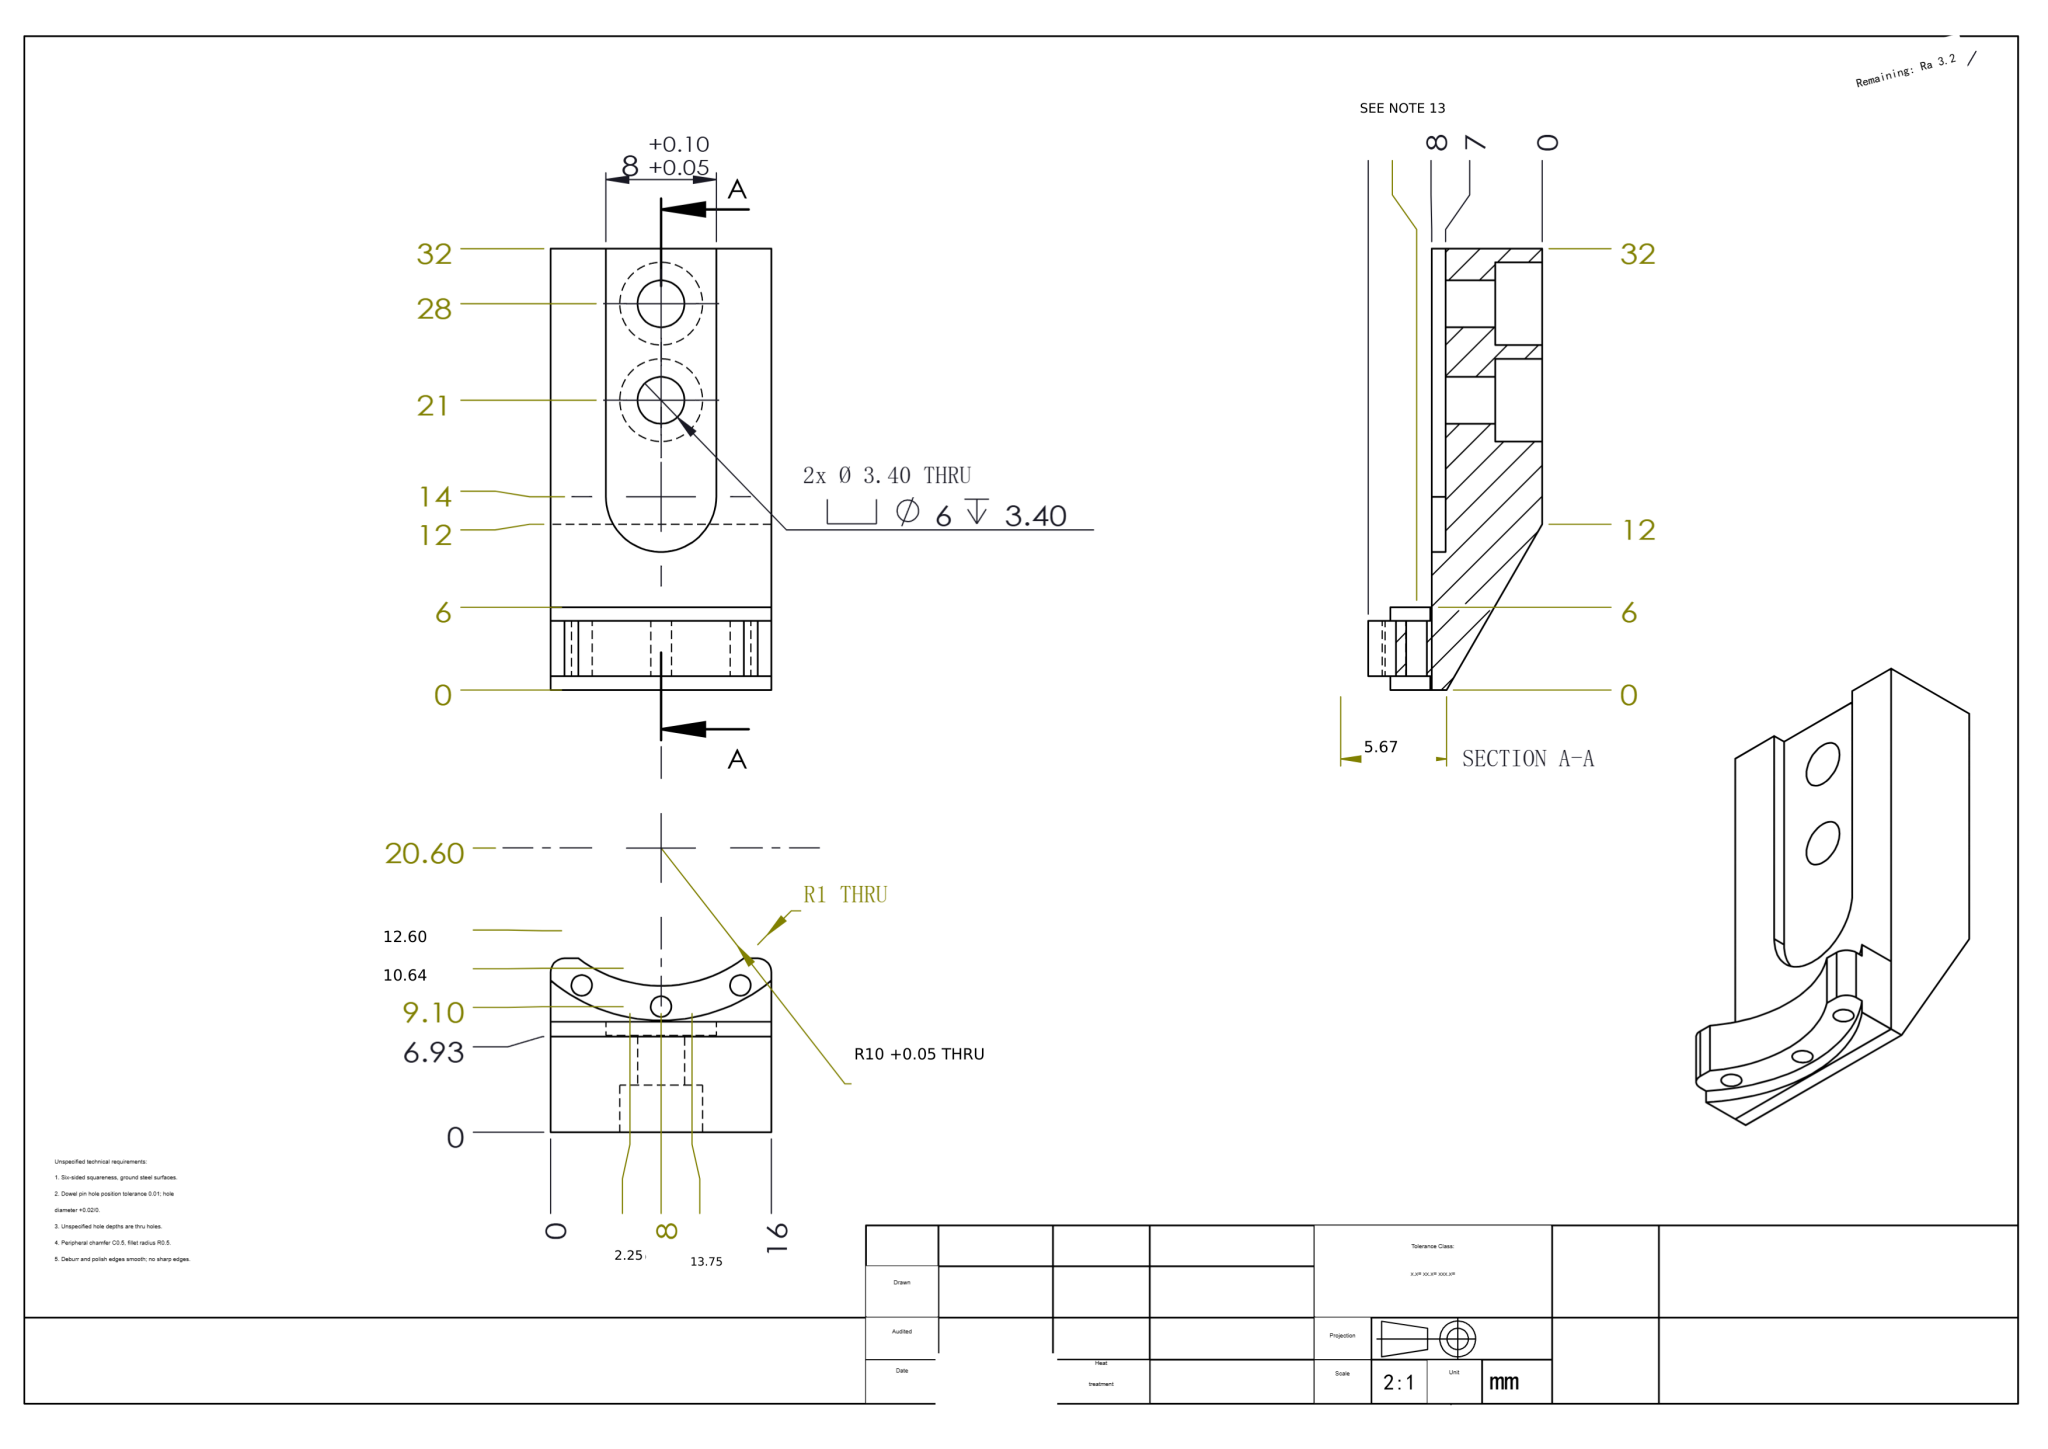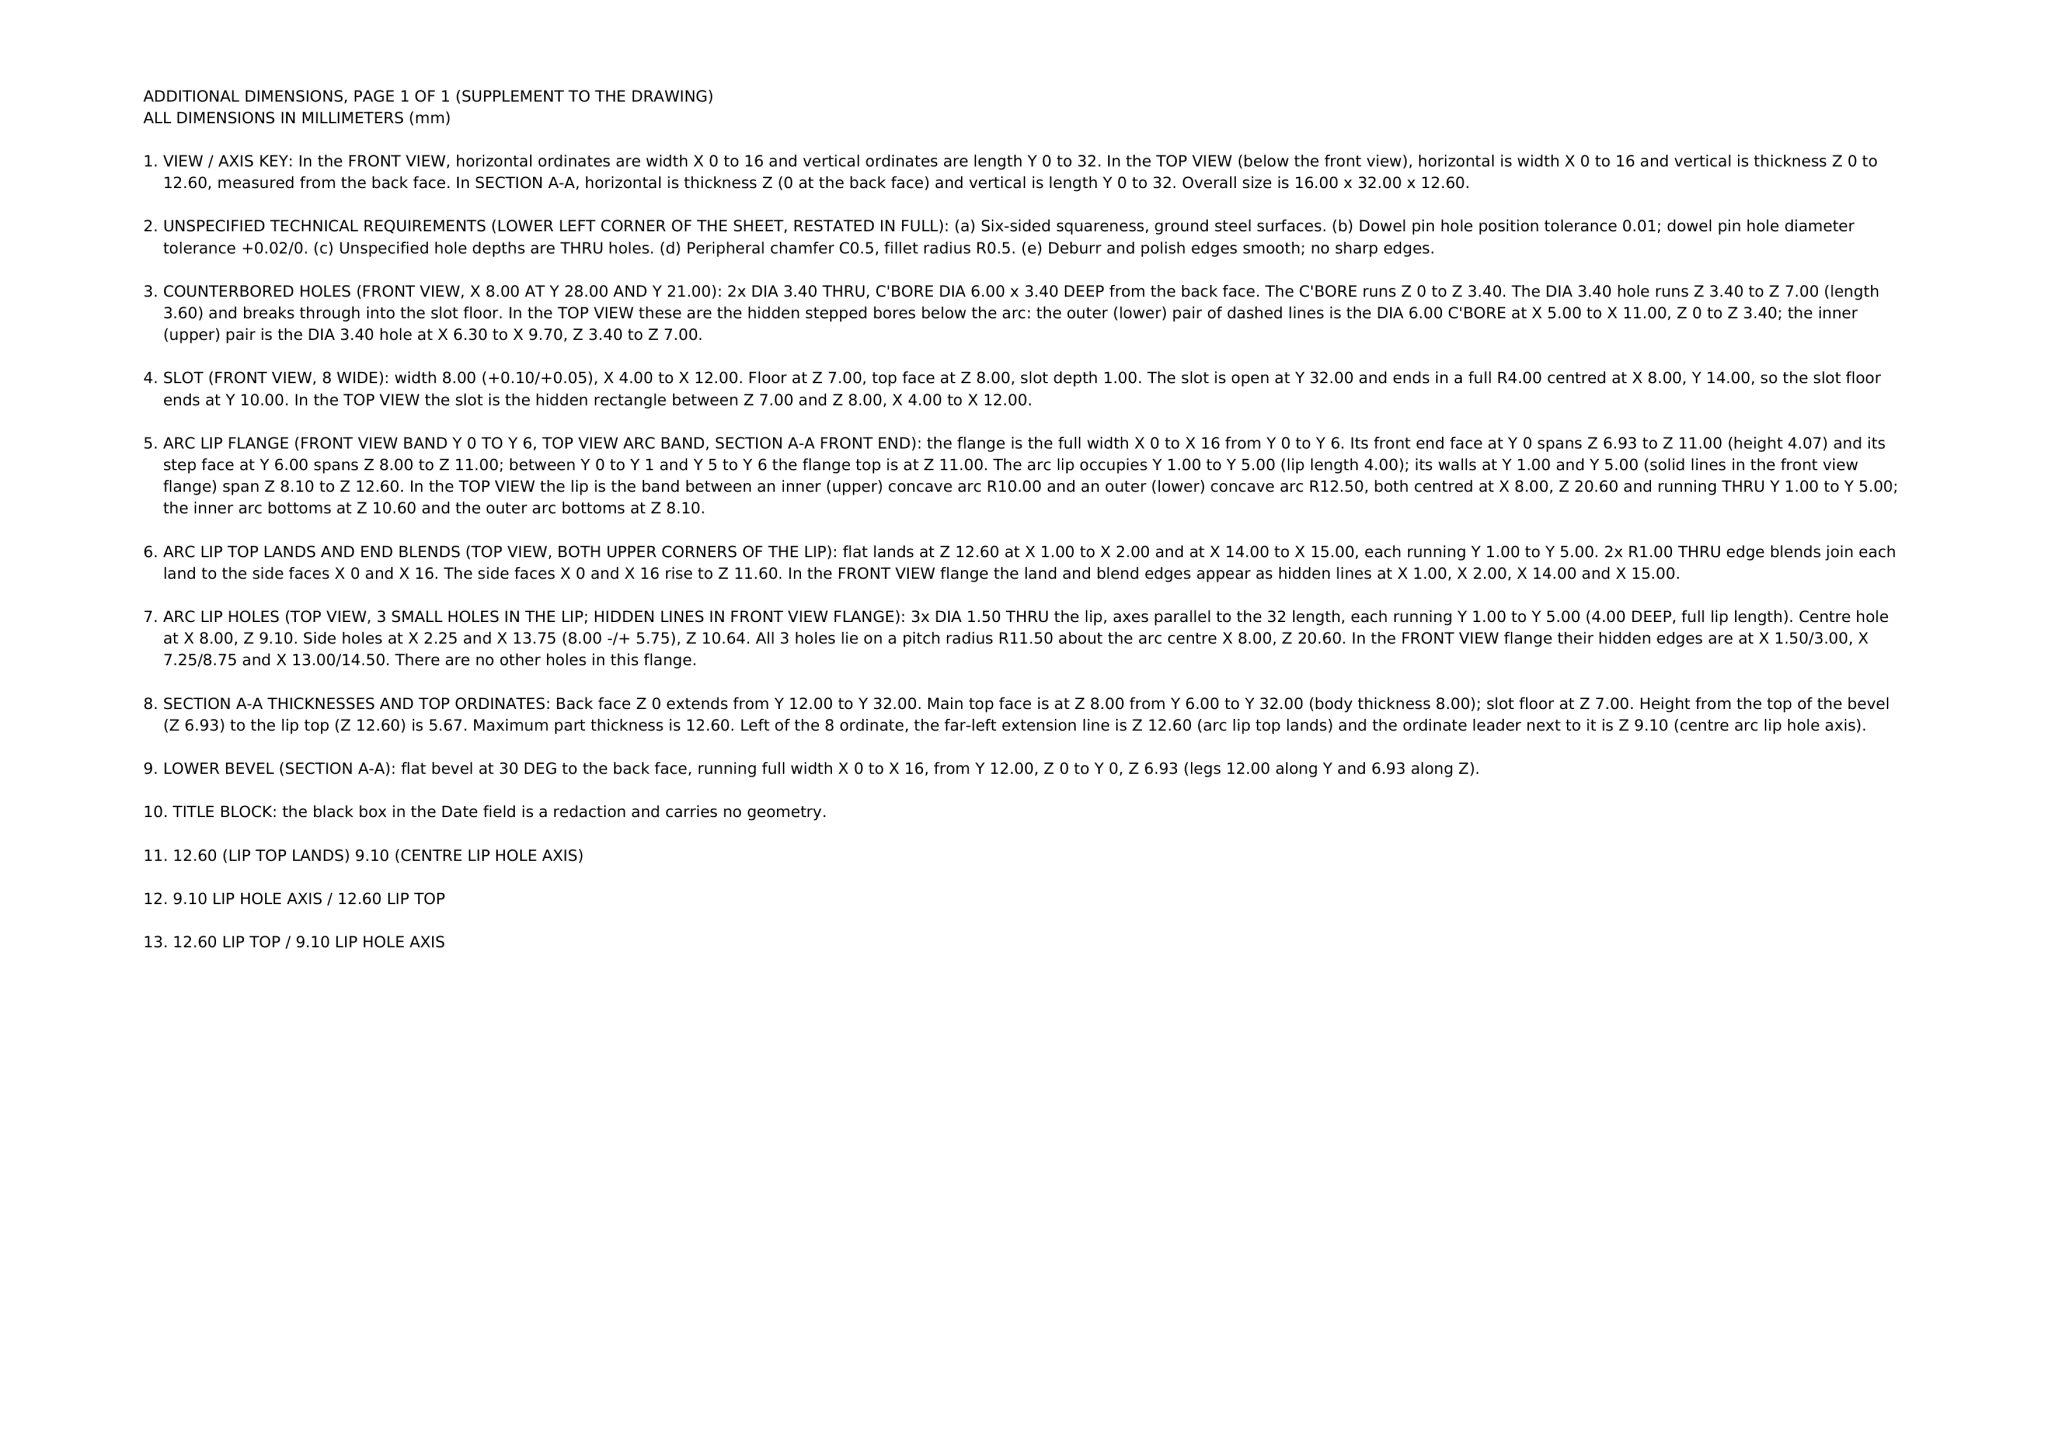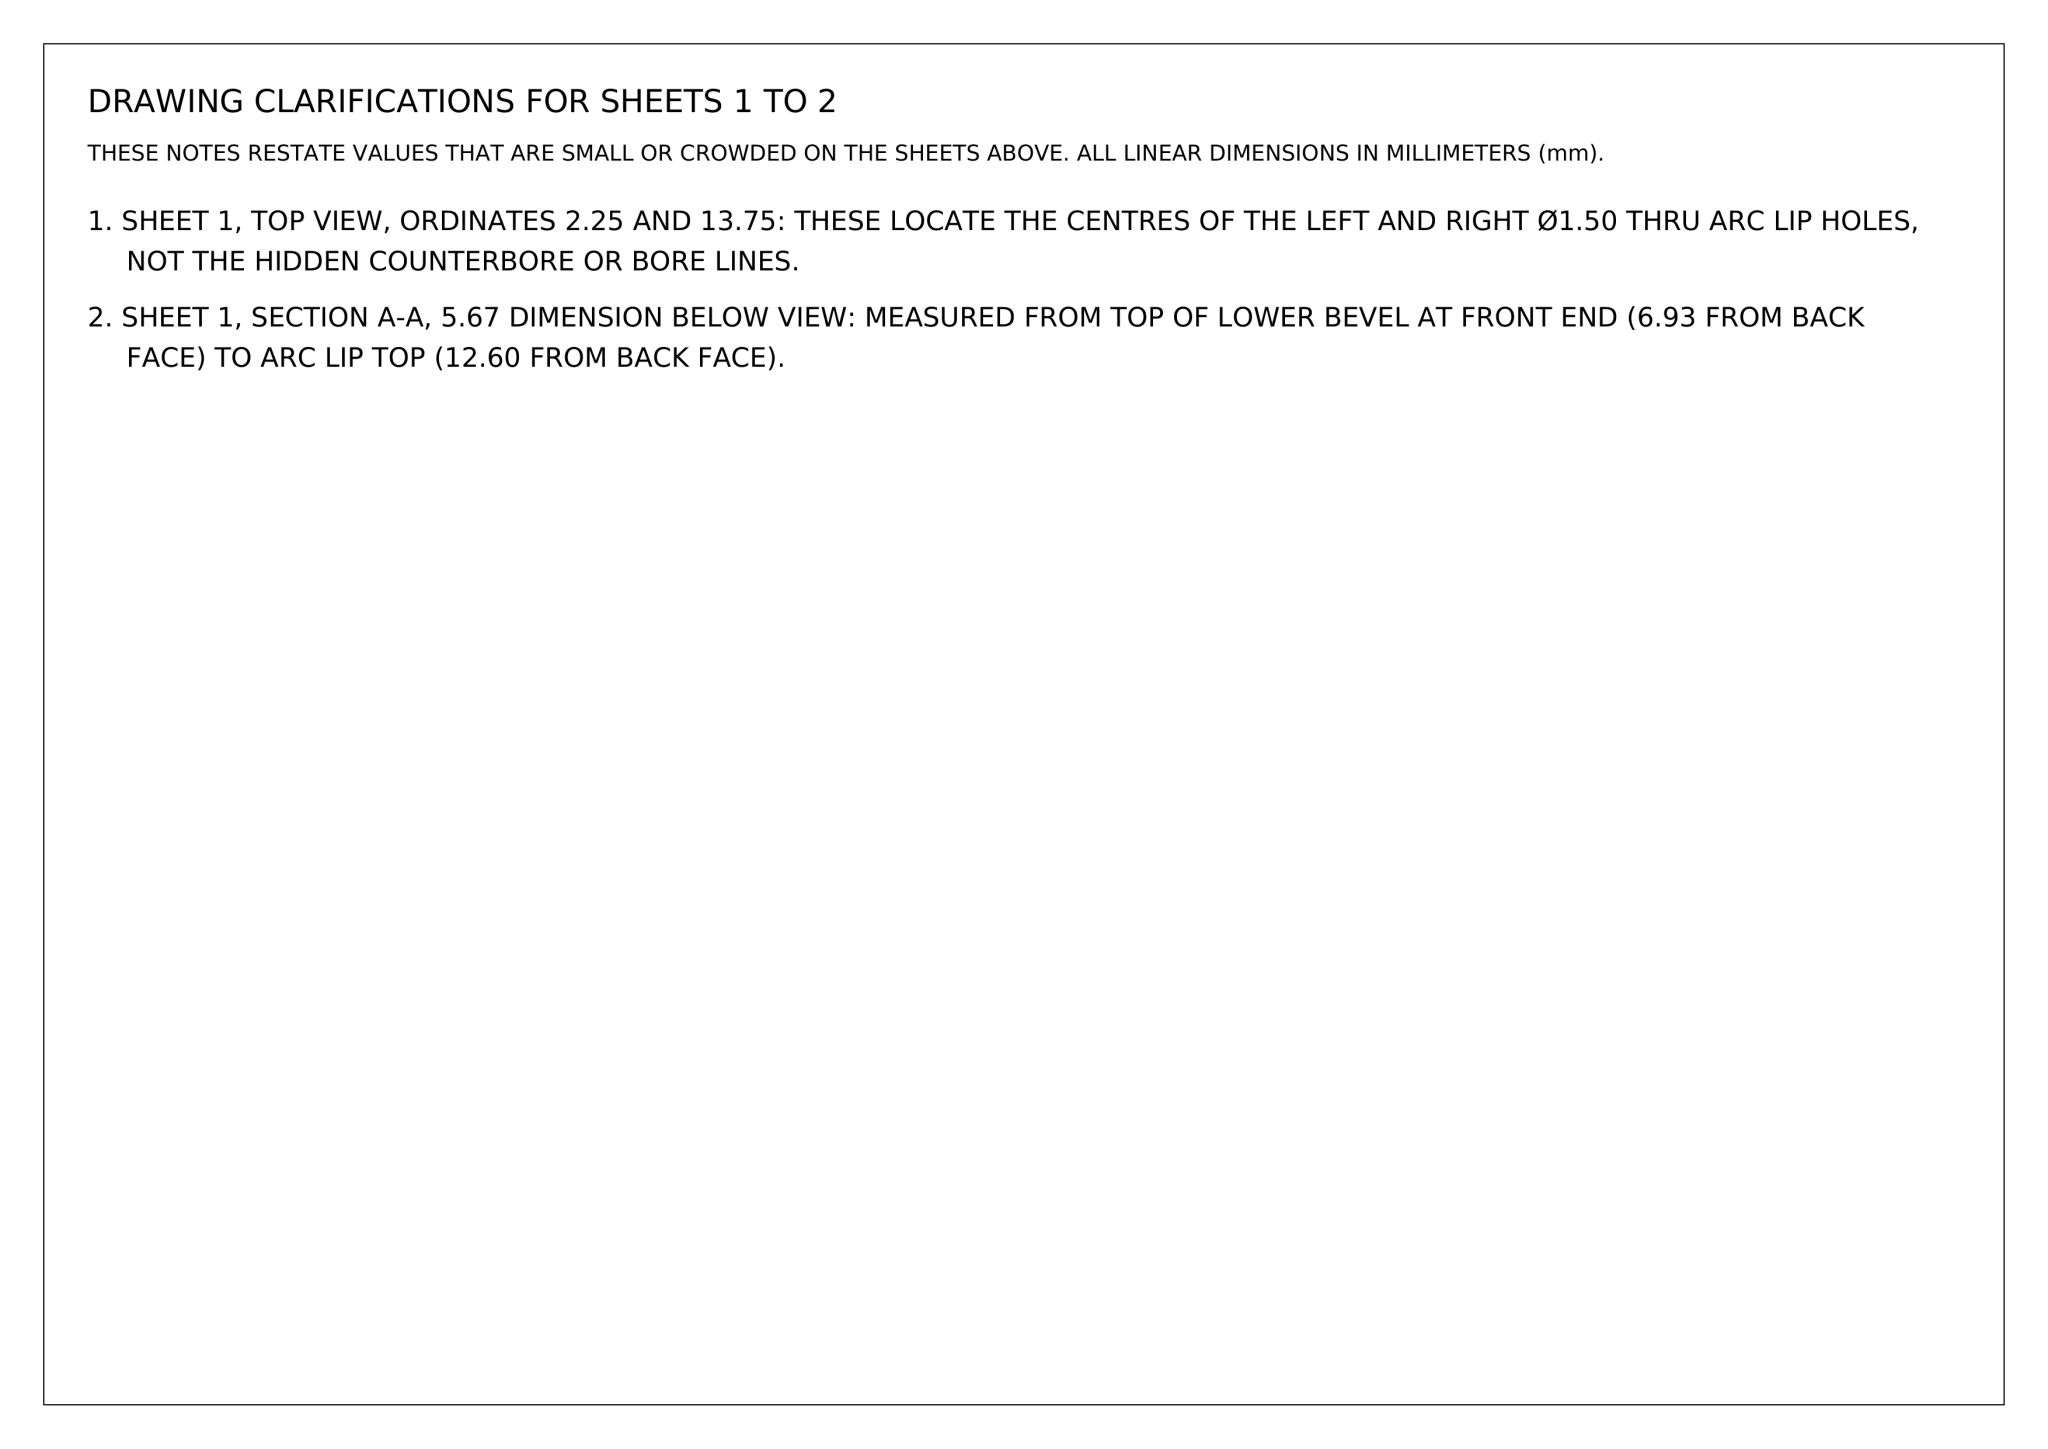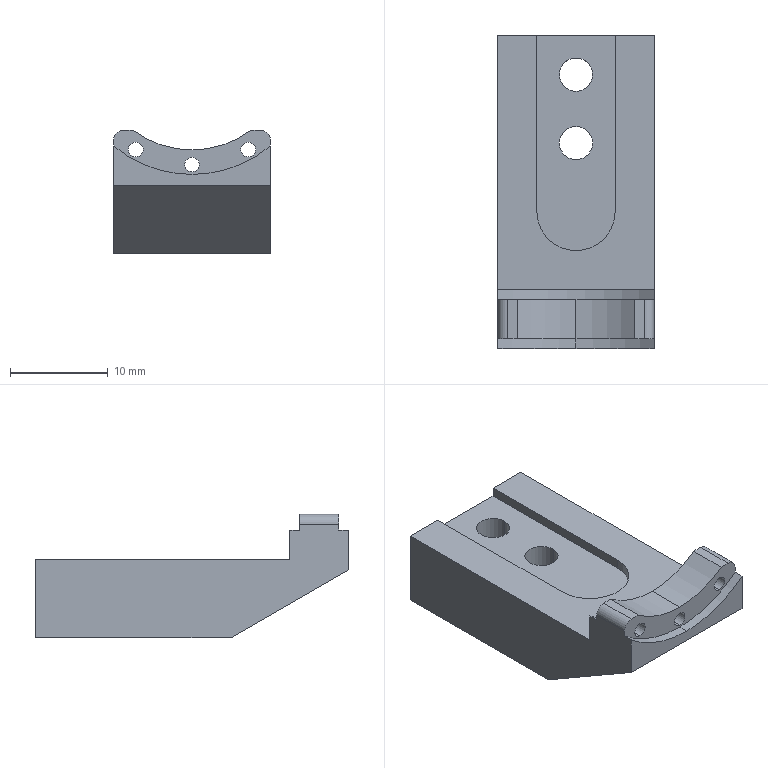Part | NX | mm | 1 solid | 39 faces | box 16 x 32 x 12.6 mm | volume 3243 mm3 | cylinder 22 | plane 17 | commonest cylinder face diameters 1.5 x6 6 x4 3.4 x4 25 x3 2 x2 20 x2 8 x1